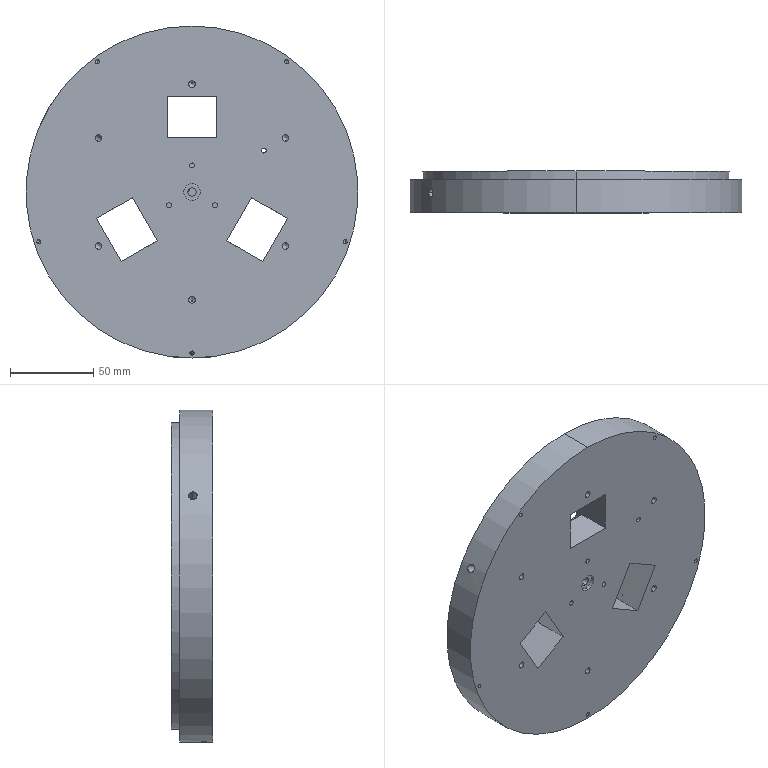Component | SolidWorks | LaserWorkingHeadCoreComponent-1 | 1 solid | 229 faces | volume 681917 mm3 | cylinder 130 | plane 72 | cone 25 | spline 2 | commonest cylinder face diameters 3 x48 4 x24 2 x18 5 x18 2.5 x10 8 x4 6.5 x2 10 x2